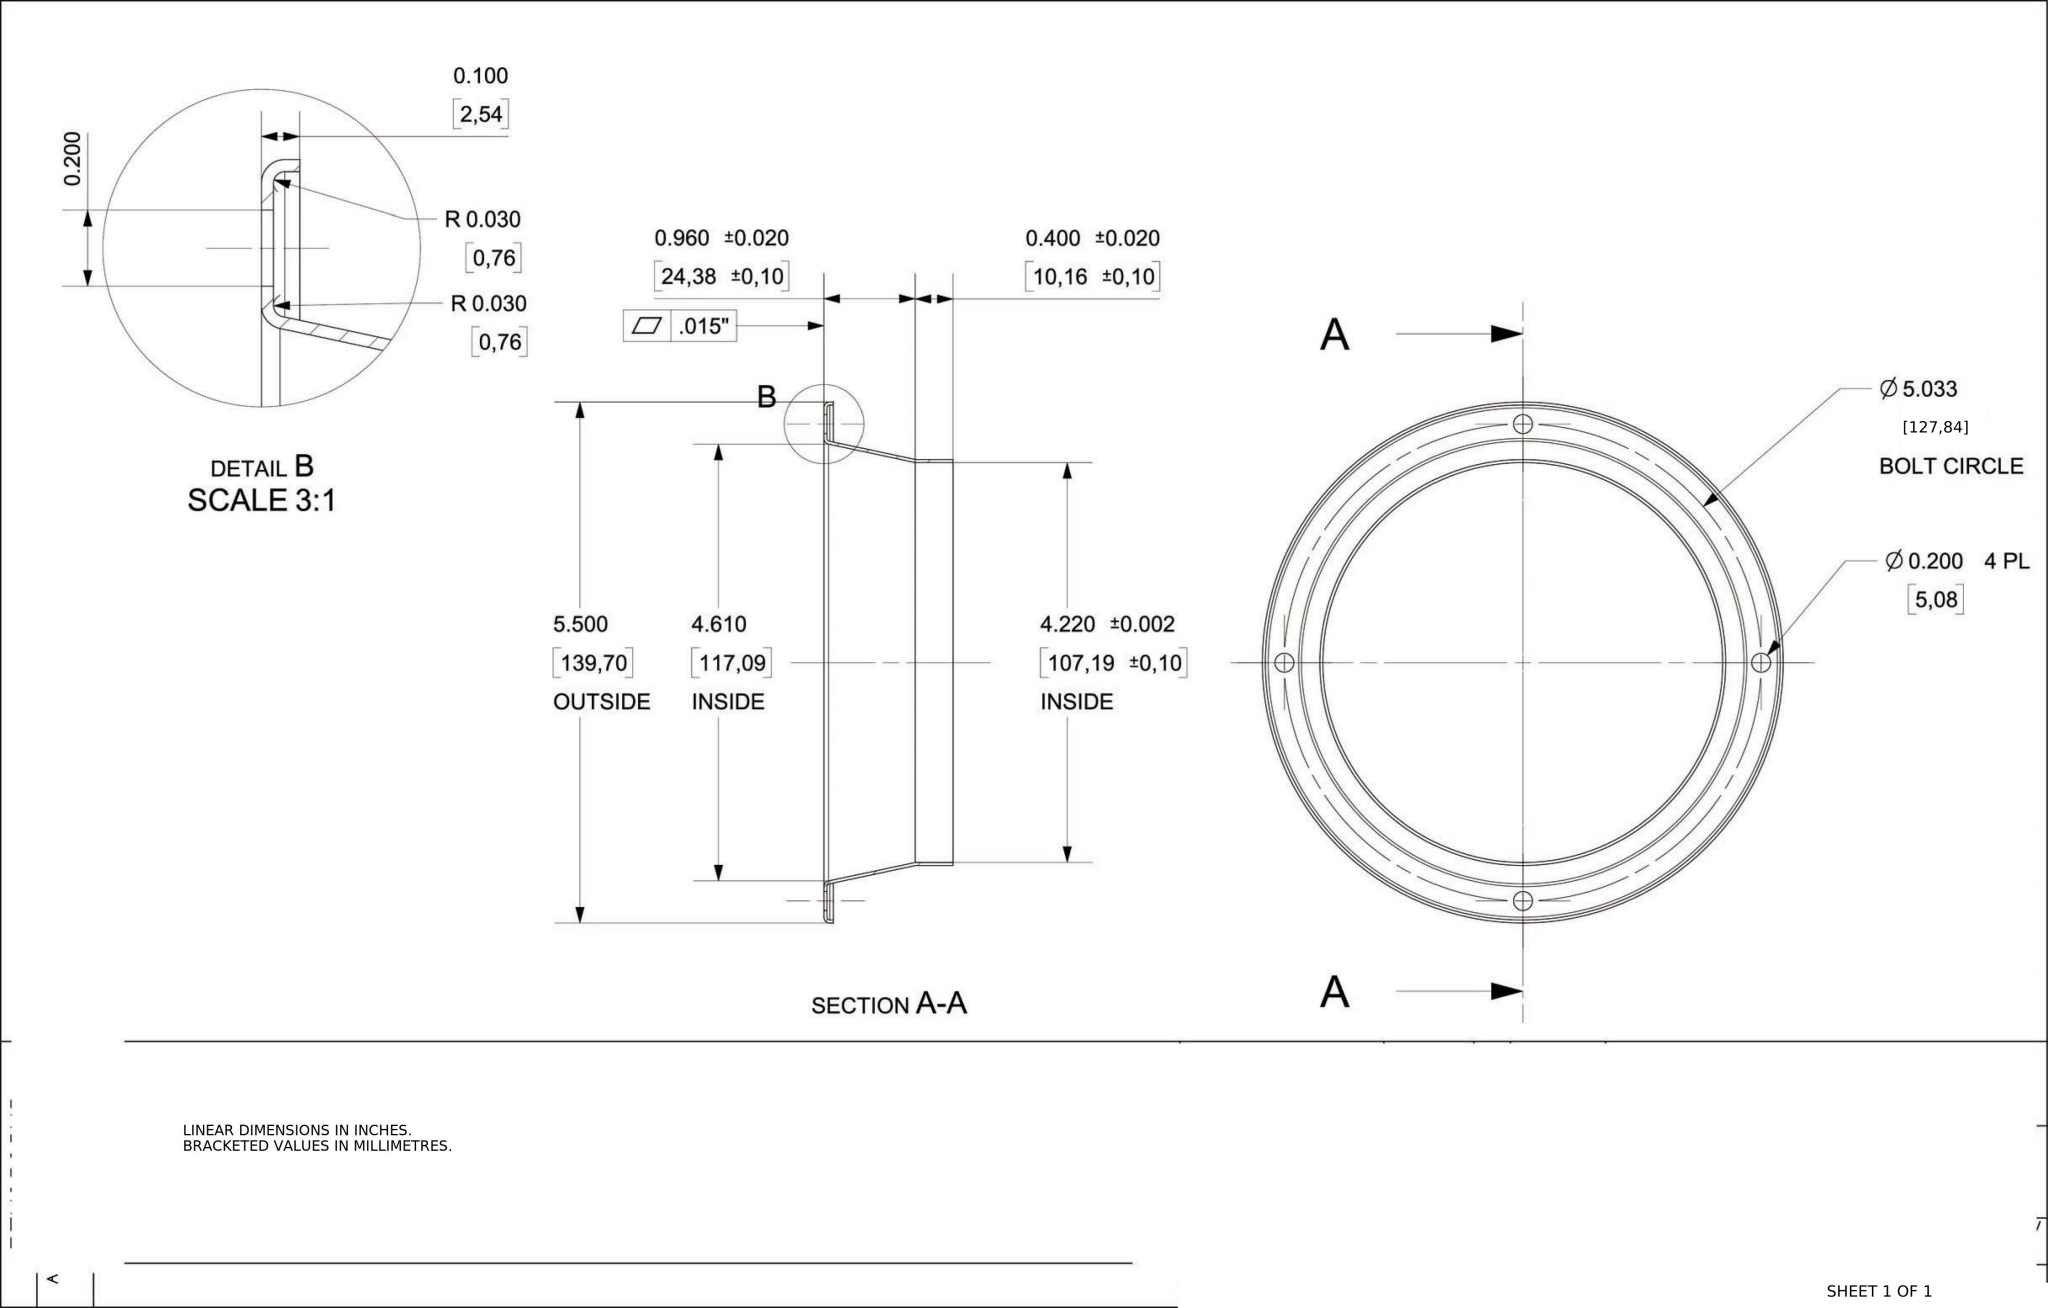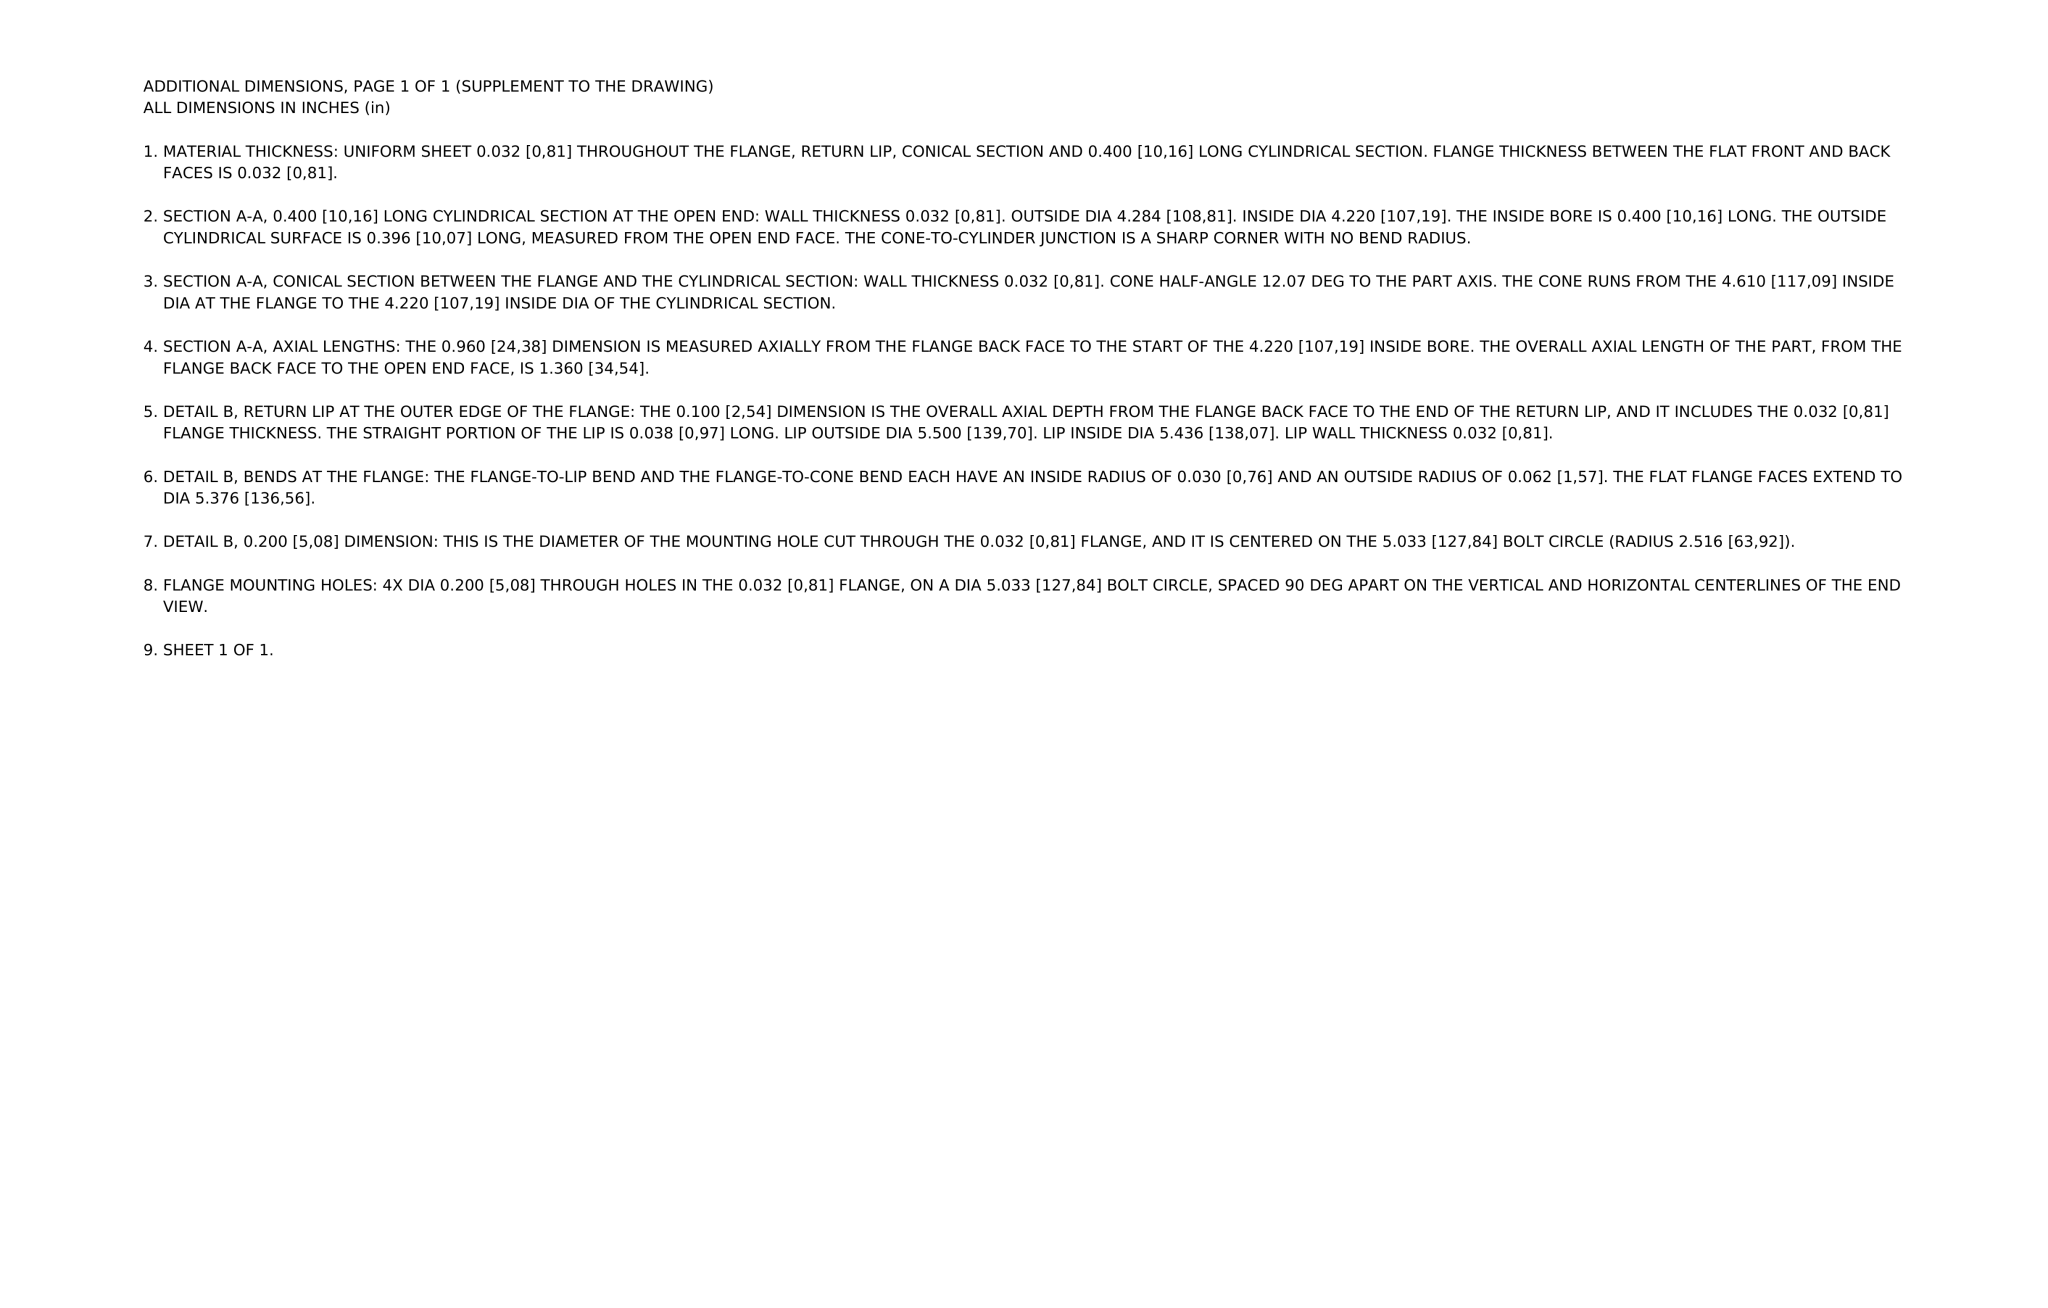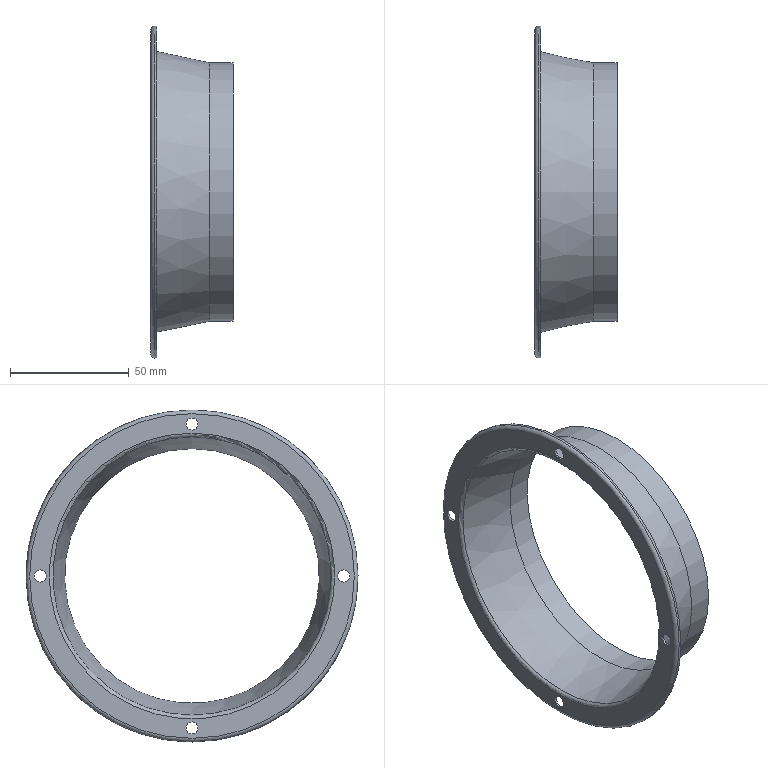Part | NX | mm | 1 solid | 18 faces | box 34.54 x 139.7 x 139.7 mm | volume 13664 mm3 | cylinder 8 | torus 4 | plane 3 | cone 3 | commonest cylinder face diameters 5.08 x4 139.7 x1 138.074 x1 108.814 x1 107.188 x1
STEP:
#1=VALUE_REPRESENTATION_ITEM('',COUNT_MEASURE(0.));
#2=(LENGTH_UNIT()NAMED_UNIT(*)SI_UNIT(.MILLI.,.METRE.));
#3=LENGTH_MEASURE_WITH_UNIT(LENGTH_MEASURE(25.4),#2);
#4=DIMENSIONAL_EXPONENTS(1.,0.,0.,0.,0.,0.,0.);
#5=(CONVERSION_BASED_UNIT('',#3)LENGTH_UNIT()NAMED_UNIT(#4));
#6=UNCERTAINTY_MEASURE_WITH_UNIT(LENGTH_MEASURE(0.002),#5,'','');
#7=(NAMED_UNIT(*)PLANE_ANGLE_UNIT()SI_UNIT($,.RADIAN.));
#8=PLANE_ANGLE_MEASURE_WITH_UNIT(PLANE_ANGLE_MEASURE(0.01745),#7);
#9=DIMENSIONAL_EXPONENTS(0.,0.,0.,0.,0.,0.,0.);
#10=(CONVERSION_BASED_UNIT('',#8)NAMED_UNIT(#9)PLANE_ANGLE_UNIT());
#11=(NAMED_UNIT(*)SI_UNIT($,.STERADIAN.)SOLID_ANGLE_UNIT());
#12=(GEOMETRIC_REPRESENTATION_CONTEXT(3)GLOBAL_UNCERTAINTY_ASSIGNED_CONTEXT((#6))GLOBAL_UNIT_ASSIGNED_CONTEXT((#5,#10,#11))REPRESENTATION_CONTEXT('',''));
#13=REPRESENTATION('',(#1),#12);
#14=VALUE_REPRESENTATION_ITEM('',COUNT_MEASURE(0.));
#15=REPRESENTATION('',(#14),#12);
#16=CARTESIAN_POINT('',(0.,0.,0.));
#17=DIRECTION('',(0.,0.,1.));
#18=DIRECTION('',(1.,0.,0.));
#19=AXIS2_PLACEMENT_3D('',#16,#17,#18);
#20=SHAPE_REPRESENTATION('',(#19),#12);
#21=CARTESIAN_POINT('',(-5.31,0.,2.688));
#22=VERTEX_POINT('',#21);
#23=CARTESIAN_POINT('',(-5.31,0.,-0.));
#24=DIRECTION('',(-1.,0.,0.));
#25=DIRECTION('',(0.,0.,1.));
#26=AXIS2_PLACEMENT_3D('',#23,#24,#25);
#27=CIRCLE('',#26,2.688);
#28=EDGE_CURVE('',#22,#22,#27,.T.);
#29=ORIENTED_EDGE('',*,*,#28,.T.);
#30=EDGE_LOOP('',(#29));
#31=FACE_BOUND('',#30,.T.);
#32=CARTESIAN_POINT('',(-5.31,0.,2.366));
#33=VERTEX_POINT('',#32);
#34=CARTESIAN_POINT('',(-5.31,0.,-0.));
#35=DIRECTION('',(1.,0.,0.));
#36=DIRECTION('',(0.,0.,1.));
#37=AXIS2_PLACEMENT_3D('',#34,#35,#36);
#38=CIRCLE('',#37,2.366);
#39=EDGE_CURVE('',#33,#33,#38,.T.);
#40=ORIENTED_EDGE('',*,*,#39,.T.);
#41=EDGE_LOOP('',(#40));
#42=FACE_BOUND('',#41,.T.);
#43=CARTESIAN_POINT('',(-5.31,-2.517,0.1));
#44=VERTEX_POINT('',#43);
#45=CARTESIAN_POINT('',(-5.31,-2.517,-0.));
#46=DIRECTION('',(-1.,0.,0.));
#47=DIRECTION('',(0.,0.,1.));
#48=AXIS2_PLACEMENT_3D('',#45,#46,#47);
#49=CIRCLE('',#48,0.1);
#50=EDGE_CURVE('',#44,#44,#49,.T.);
#51=ORIENTED_EDGE('',*,*,#50,.F.);
#52=EDGE_LOOP('',(#51));
#53=FACE_BOUND('',#52,.T.);
#54=CARTESIAN_POINT('',(-5.31,0.,2.617));
#55=VERTEX_POINT('',#54);
#56=CARTESIAN_POINT('',(-5.31,0.,2.517));
#57=DIRECTION('',(-1.,0.,0.));
#58=DIRECTION('',(0.,0.,1.));
#59=AXIS2_PLACEMENT_3D('',#56,#57,#58);
#60=CIRCLE('',#59,0.1);
#61=EDGE_CURVE('',#55,#55,#60,.T.);
#62=ORIENTED_EDGE('',*,*,#61,.F.);
#63=EDGE_LOOP('',(#62));
#64=FACE_BOUND('',#63,.T.);
#65=CARTESIAN_POINT('',(-5.31,2.517,0.1));
#66=VERTEX_POINT('',#65);
#67=CARTESIAN_POINT('',(-5.31,2.517,-0.));
#68=DIRECTION('',(-1.,0.,0.));
#69=DIRECTION('',(0.,0.,1.));
#70=AXIS2_PLACEMENT_3D('',#67,#68,#69);
#71=CIRCLE('',#70,0.1);
#72=EDGE_CURVE('',#66,#66,#71,.T.);
#73=ORIENTED_EDGE('',*,*,#72,.F.);
#74=EDGE_LOOP('',(#73));
#75=FACE_BOUND('',#74,.T.);
#76=CARTESIAN_POINT('',(-5.31,0.,-2.417));
#77=VERTEX_POINT('',#76);
#78=CARTESIAN_POINT('',(-5.31,0.,-2.517));
#79=DIRECTION('',(-1.,0.,0.));
#80=DIRECTION('',(0.,0.,1.));
#81=AXIS2_PLACEMENT_3D('',#78,#79,#80);
#82=CIRCLE('',#81,0.1);
#83=EDGE_CURVE('',#77,#77,#82,.T.);
#84=ORIENTED_EDGE('',*,*,#83,.F.);
#85=EDGE_LOOP('',(#84));
#86=FACE_BOUND('',#85,.T.);
#87=CARTESIAN_POINT('',(-5.31,0.,-2.315));
#88=DIRECTION('',(-1.,0.,0.));
#89=DIRECTION('',(0.,0.,1.));
#90=AXIS2_PLACEMENT_3D('',#87,#88,#89);
#91=PLANE('',#90);
#92=ADVANCED_FACE('',(#31,#42,#53,#64,#75,#86),#91,.T.);
#93=CARTESIAN_POINT('',(-5.248,0.,2.75));
#94=VERTEX_POINT('',#93);
#95=CARTESIAN_POINT('',(-5.248,0.,-0.));
#96=DIRECTION('',(1.,0.,0.));
#97=DIRECTION('',(0.,0.,1.));
#98=AXIS2_PLACEMENT_3D('',#95,#96,#97);
#99=CIRCLE('',#98,2.75);
#100=EDGE_CURVE('',#94,#94,#99,.T.);
#101=ORIENTED_EDGE('',*,*,#100,.T.);
#102=EDGE_LOOP('',(#101));
#103=FACE_BOUND('',#102,.T.);
#104=CARTESIAN_POINT('',(-5.21,-0.,-2.75));
#105=VERTEX_POINT('',#104);
#106=CARTESIAN_POINT('',(-5.21,0.36,-2.75));
#107=CARTESIAN_POINT('',(-5.21,-0.36,-2.75));
#108=CARTESIAN_POINT('',(-5.21,-0.7198,-2.678));
#109=CARTESIAN_POINT('',(-5.21,-1.385,-2.403));
#110=CARTESIAN_POINT('',(-5.21,-1.69,-2.199));
#111=CARTESIAN_POINT('',(-5.21,-2.199,-1.69));
#112=CARTESIAN_POINT('',(-5.21,-2.403,-1.385));
#113=CARTESIAN_POINT('',(-5.21,-2.678,-0.7198));
#114=CARTESIAN_POINT('',(-5.21,-2.75,-0.36));
#115=CARTESIAN_POINT('',(-5.21,-2.75,0.36));
#116=CARTESIAN_POINT('',(-5.21,-2.678,0.7198));
#117=CARTESIAN_POINT('',(-5.21,-2.403,1.385));
#118=CARTESIAN_POINT('',(-5.21,-2.199,1.69));
#119=CARTESIAN_POINT('',(-5.21,-1.69,2.199));
#120=CARTESIAN_POINT('',(-5.21,-1.385,2.403));
#121=CARTESIAN_POINT('',(-5.21,-0.7198,2.678));
#122=CARTESIAN_POINT('',(-5.21,-0.36,2.75));
#123=CARTESIAN_POINT('',(-5.21,0.36,2.75));
#124=CARTESIAN_POINT('',(-5.21,0.7198,2.678));
#125=CARTESIAN_POINT('',(-5.21,1.385,2.403));
#126=CARTESIAN_POINT('',(-5.21,1.69,2.199));
#127=CARTESIAN_POINT('',(-5.21,2.199,1.69));
#128=CARTESIAN_POINT('',(-5.21,2.403,1.385));
#129=CARTESIAN_POINT('',(-5.21,2.678,0.7198));
#130=CARTESIAN_POINT('',(-5.21,2.75,0.36));
#131=CARTESIAN_POINT('',(-5.21,2.75,-0.36));
#132=CARTESIAN_POINT('',(-5.21,2.678,-0.7198));
#133=CARTESIAN_POINT('',(-5.21,2.403,-1.385));
#134=CARTESIAN_POINT('',(-5.21,2.199,-1.69));
#135=CARTESIAN_POINT('',(-5.21,1.69,-2.199));
#136=CARTESIAN_POINT('',(-5.21,1.385,-2.403));
#137=CARTESIAN_POINT('',(-5.21,0.7198,-2.678));
#138=CARTESIAN_POINT('',(-5.21,0.36,-2.75));
#139=CARTESIAN_POINT('',(-5.21,-0.36,-2.75));
#140=B_SPLINE_CURVE_WITH_KNOTS('',3,(#106,#107,#108,#109,#110,#111,#112,#113,#114,#115,#116,#117,#118,#119,#120,#121,#122,#123,#124,#125,#126,#127,#128,#129,#130,#131,#132,#133,#134,#135,#136,#137,#138,#139),.UNSPECIFIED.,.T.,.F.,(2,2,2,2,2,2,2,2,2,2,2,2,2,2,2,2,2,2,2),(-0.0625,0.,0.0625,0.125,0.1875,0.25,0.3125,0.375,0.4375,0.5,0.5625,0.625,0.6875,0.75,0.8125,0.875,0.9375,1.,1.062),.UNSPECIFIED.);
#141=EDGE_CURVE('',#105,#105,#140,.T.);
#142=ORIENTED_EDGE('',*,*,#141,.T.);
#143=EDGE_LOOP('',(#142));
#144=FACE_BOUND('',#143,.T.);
#145=CARTESIAN_POINT('',(-0.28,0.,-0.));
#146=DIRECTION('',(-1.,0.,0.));
#147=DIRECTION('',(0.,0.,1.));
#148=AXIS2_PLACEMENT_3D('',#145,#146,#147);
#149=CYLINDRICAL_SURFACE('',#148,2.75);
#150=ADVANCED_FACE('',(#103,#144),#149,.T.);
#151=CARTESIAN_POINT('',(-5.21,0.,2.718));
#152=VERTEX_POINT('',#151);
#153=CARTESIAN_POINT('',(-5.21,0.,-0.));
#154=DIRECTION('',(-1.,0.,0.));
#155=DIRECTION('',(0.,0.,1.));
#156=AXIS2_PLACEMENT_3D('',#153,#154,#155);
#157=CIRCLE('',#156,2.718);
#158=EDGE_CURVE('',#152,#152,#157,.T.);
#159=ORIENTED_EDGE('',*,*,#158,.T.);
#160=EDGE_LOOP('',(#159));
#161=FACE_BOUND('',#160,.T.);
#162=ORIENTED_EDGE('',*,*,#141,.F.);
#163=EDGE_LOOP('',(#162));
#164=FACE_BOUND('',#163,.T.);
#165=CARTESIAN_POINT('',(-5.21,0.,-0.));
#166=DIRECTION('',(1.,0.,0.));
#167=DIRECTION('',(0.,0.,-1.));
#168=AXIS2_PLACEMENT_3D('',#165,#166,#167);
#169=CONICAL_SURFACE('',#168,2.75,89.597);
#170=ADVANCED_FACE('',(#161,#164),#169,.F.);
#171=CARTESIAN_POINT('',(-5.248,0.,-2.718));
#172=VERTEX_POINT('',#171);
#173=CARTESIAN_POINT('',(-5.248,0.,-0.));
#174=DIRECTION('',(-1.,0.,0.));
#175=DIRECTION('',(0.,0.,-1.));
#176=AXIS2_PLACEMENT_3D('',#173,#174,#175);
#177=CIRCLE('',#176,2.718);
#178=EDGE_CURVE('',#172,#172,#177,.T.);
#179=ORIENTED_EDGE('',*,*,#178,.T.);
#180=EDGE_LOOP('',(#179));
#181=FACE_BOUND('',#180,.T.);
#182=ORIENTED_EDGE('',*,*,#158,.F.);
#183=EDGE_LOOP('',(#182));
#184=FACE_BOUND('',#183,.T.);
#185=CARTESIAN_POINT('',(-0.28,0.,-0.));
#186=DIRECTION('',(-1.,0.,0.));
#187=DIRECTION('',(0.,0.,1.));
#188=AXIS2_PLACEMENT_3D('',#185,#186,#187);
#189=CYLINDRICAL_SURFACE('',#188,2.718);
#190=ADVANCED_FACE('',(#181,#184),#189,.F.);
#191=CARTESIAN_POINT('',(-5.278,0.,-2.688));
#192=VERTEX_POINT('',#191);
#193=CARTESIAN_POINT('',(-5.278,0.,-0.));
#194=DIRECTION('',(1.,0.,0.));
#195=DIRECTION('',(0.,0.,-1.));
#196=AXIS2_PLACEMENT_3D('',#193,#194,#195);
#197=CIRCLE('',#196,2.688);
#198=EDGE_CURVE('',#192,#192,#197,.T.);
#199=ORIENTED_EDGE('',*,*,#198,.T.);
#200=EDGE_LOOP('',(#199));
#201=FACE_BOUND('',#200,.T.);
#202=CARTESIAN_POINT('',(-5.278,-2.517,0.1));
#203=VERTEX_POINT('',#202);
#204=CARTESIAN_POINT('',(-5.278,-2.517,-0.));
#205=DIRECTION('',(-1.,0.,0.));
#206=DIRECTION('',(0.,0.,1.));
#207=AXIS2_PLACEMENT_3D('',#204,#205,#206);
#208=CIRCLE('',#207,0.1);
#209=EDGE_CURVE('',#203,#203,#208,.T.);
#210=ORIENTED_EDGE('',*,*,#209,.T.);
#211=EDGE_LOOP('',(#210));
#212=FACE_BOUND('',#211,.T.);
#213=CARTESIAN_POINT('',(-5.278,0.,2.617));
#214=VERTEX_POINT('',#213);
#215=CARTESIAN_POINT('',(-5.278,0.,2.517));
#216=DIRECTION('',(-1.,0.,0.));
#217=DIRECTION('',(0.,0.,1.));
#218=AXIS2_PLACEMENT_3D('',#215,#216,#217);
#219=CIRCLE('',#218,0.1);
#220=EDGE_CURVE('',#214,#214,#219,.T.);
#221=ORIENTED_EDGE('',*,*,#220,.T.);
#222=EDGE_LOOP('',(#221));
#223=FACE_BOUND('',#222,.T.);
#224=CARTESIAN_POINT('',(-5.278,2.517,0.1));
#225=VERTEX_POINT('',#224);
#226=CARTESIAN_POINT('',(-5.278,2.517,-0.));
#227=DIRECTION('',(-1.,0.,0.));
#228=DIRECTION('',(0.,0.,1.));
#229=AXIS2_PLACEMENT_3D('',#226,#227,#228);
#230=CIRCLE('',#229,0.1);
#231=EDGE_CURVE('',#225,#225,#230,.T.);
#232=ORIENTED_EDGE('',*,*,#231,.T.);
#233=EDGE_LOOP('',(#232));
#234=FACE_BOUND('',#233,.T.);
#235=CARTESIAN_POINT('',(-5.278,0.,-2.417));
#236=VERTEX_POINT('',#235);
#237=CARTESIAN_POINT('',(-5.278,0.,-2.517));
#238=DIRECTION('',(-1.,0.,0.));
#239=DIRECTION('',(0.,0.,1.));
#240=AXIS2_PLACEMENT_3D('',#237,#238,#239);
#241=CIRCLE('',#240,0.1);
#242=EDGE_CURVE('',#236,#236,#241,.T.);
#243=ORIENTED_EDGE('',*,*,#242,.T.);
#244=EDGE_LOOP('',(#243));
#245=FACE_BOUND('',#244,.T.);
#246=CARTESIAN_POINT('',(-5.278,0.,2.366));
#247=VERTEX_POINT('',#246);
#248=CARTESIAN_POINT('',(-5.278,0.,-0.));
#249=DIRECTION('',(-1.,0.,0.));
#250=DIRECTION('',(0.,0.,1.));
#251=AXIS2_PLACEMENT_3D('',#248,#249,#250);
#252=CIRCLE('',#251,2.366);
#253=EDGE_CURVE('',#247,#247,#252,.T.);
#254=ORIENTED_EDGE('',*,*,#253,.T.);
#255=EDGE_LOOP('',(#254));
#256=FACE_BOUND('',#255,.T.);
#257=CARTESIAN_POINT('',(-5.278,0.,-2.718));
#258=DIRECTION('',(1.,0.,0.));
#259=DIRECTION('',(0.,0.,-1.));
#260=AXIS2_PLACEMENT_3D('',#257,#258,#259);
#261=PLANE('',#260);
#262=ADVANCED_FACE('',(#201,#212,#223,#234,#245,#256),#261,.T.);
#263=CARTESIAN_POINT('',(-5.254,0.,2.336));
#264=VERTEX_POINT('',#263);
#265=CARTESIAN_POINT('',(-5.254,0.,-0.));
#266=DIRECTION('',(-1.,0.,0.));
#267=DIRECTION('',(0.,0.,1.));
#268=AXIS2_PLACEMENT_3D('',#265,#266,#267);
#269=CIRCLE('',#268,2.336);
#270=EDGE_CURVE('',#264,#264,#269,.T.);
#271=ORIENTED_EDGE('',*,*,#270,.T.);
#272=EDGE_LOOP('',(#271));
#273=FACE_BOUND('',#272,.T.);
#274=ORIENTED_EDGE('',*,*,#253,.F.);
#275=EDGE_LOOP('',(#274));
#276=FACE_BOUND('',#275,.T.);
#277=CARTESIAN_POINT('',(-5.248,0.,-0.));
#278=DIRECTION('',(-1.,0.,0.));
#279=DIRECTION('',(0.,0.,1.));
#280=AXIS2_PLACEMENT_3D('',#277,#278,#279);
#281=TOROIDAL_SURFACE('',#280,2.366,0.03);
#282=ADVANCED_FACE('',(#273,#276),#281,.F.);
#283=CARTESIAN_POINT('',(-4.347,0.,2.142));
#284=VERTEX_POINT('',#283);
#285=CARTESIAN_POINT('',(-4.347,0.,-0.));
#286=DIRECTION('',(-1.,0.,0.));
#287=DIRECTION('',(0.,0.,1.));
#288=AXIS2_PLACEMENT_3D('',#285,#286,#287);
#289=CIRCLE('',#288,2.142);
#290=EDGE_CURVE('',#284,#284,#289,.T.);
#291=ORIENTED_EDGE('',*,*,#290,.T.);
#292=EDGE_LOOP('',(#291));
#293=FACE_BOUND('',#292,.T.);
#294=ORIENTED_EDGE('',*,*,#270,.F.);
#295=EDGE_LOOP('',(#294));
#296=FACE_BOUND('',#295,.T.);
#297=CARTESIAN_POINT('',(-5.254,0.,-0.));
#298=DIRECTION('',(-1.,0.,0.));
#299=DIRECTION('',(-0.,0.,1.));
#300=AXIS2_PLACEMENT_3D('',#297,#298,#299);
#301=CONICAL_SURFACE('',#300,2.336,12.075);
#302=ADVANCED_FACE('',(#293,#296),#301,.T.);
#303=CARTESIAN_POINT('',(-3.95,0.,2.142));
#304=VERTEX_POINT('',#303);
#305=CARTESIAN_POINT('',(-3.95,0.,-0.));
#306=DIRECTION('',(-1.,0.,0.));
#307=DIRECTION('',(0.,0.,1.));
#308=AXIS2_PLACEMENT_3D('',#305,#306,#307);
#309=CIRCLE('',#308,2.142);
#310=EDGE_CURVE('',#304,#304,#309,.T.);
#311=ORIENTED_EDGE('',*,*,#310,.T.);
#312=EDGE_LOOP('',(#311));
#313=FACE_BOUND('',#312,.T.);
#314=ORIENTED_EDGE('',*,*,#290,.F.);
#315=EDGE_LOOP('',(#314));
#316=FACE_BOUND('',#315,.T.);
#317=CARTESIAN_POINT('',(-0.28,0.,-0.));
#318=DIRECTION('',(-1.,0.,0.));
#319=DIRECTION('',(0.,0.,1.));
#320=AXIS2_PLACEMENT_3D('',#317,#318,#319);
#321=CYLINDRICAL_SURFACE('',#320,2.142);
#322=ADVANCED_FACE('',(#313,#316),#321,.T.);
#323=CARTESIAN_POINT('',(-3.95,0.,2.11));
#324=VERTEX_POINT('',#323);
#325=CARTESIAN_POINT('',(-3.95,0.,-0.));
#326=DIRECTION('',(-1.,0.,0.));
#327=DIRECTION('',(0.,0.,1.));
#328=AXIS2_PLACEMENT_3D('',#325,#326,#327);
#329=CIRCLE('',#328,2.11);
#330=EDGE_CURVE('',#324,#324,#329,.T.);
#331=ORIENTED_EDGE('',*,*,#330,.T.);
#332=EDGE_LOOP('',(#331));
#333=FACE_BOUND('',#332,.T.);
#334=ORIENTED_EDGE('',*,*,#310,.F.);
#335=EDGE_LOOP('',(#334));
#336=FACE_BOUND('',#335,.T.);
#337=CARTESIAN_POINT('',(-3.95,0.,-2.142));
#338=DIRECTION('',(1.,0.,0.));
#339=DIRECTION('',(0.,0.,-1.));
#340=AXIS2_PLACEMENT_3D('',#337,#338,#339);
#341=PLANE('',#340);
#342=ADVANCED_FACE('',(#333,#336),#341,.T.);
#343=CARTESIAN_POINT('',(-4.35,0.,2.11));
#344=VERTEX_POINT('',#343);
#345=CARTESIAN_POINT('',(-4.35,0.,-0.));
#346=DIRECTION('',(-1.,0.,0.));
#347=DIRECTION('',(0.,0.,1.));
#348=AXIS2_PLACEMENT_3D('',#345,#346,#347);
#349=CIRCLE('',#348,2.11);
#350=EDGE_CURVE('',#344,#344,#349,.T.);
#351=ORIENTED_EDGE('',*,*,#350,.T.);
#352=EDGE_LOOP('',(#351));
#353=FACE_BOUND('',#352,.T.);
#354=ORIENTED_EDGE('',*,*,#330,.F.);
#355=EDGE_LOOP('',(#354));
#356=FACE_BOUND('',#355,.T.);
#357=CARTESIAN_POINT('',(-0.28,0.,-0.));
#358=DIRECTION('',(-1.,0.,0.));
#359=DIRECTION('',(0.,0.,1.));
#360=AXIS2_PLACEMENT_3D('',#357,#358,#359);
#361=CYLINDRICAL_SURFACE('',#360,2.11);
#362=ADVANCED_FACE('',(#353,#356),#361,.F.);
#363=CARTESIAN_POINT('',(-5.261,0.,-2.305));
#364=VERTEX_POINT('',#363);
#365=CARTESIAN_POINT('',(-5.261,0.,-0.));
#366=DIRECTION('',(-1.,0.,0.));
#367=DIRECTION('',(0.,0.,-1.));
#368=AXIS2_PLACEMENT_3D('',#365,#366,#367);
#369=CIRCLE('',#368,2.305);
#370=EDGE_CURVE('',#364,#364,#369,.T.);
#371=ORIENTED_EDGE('',*,*,#370,.T.);
#372=EDGE_LOOP('',(#371));
#373=FACE_BOUND('',#372,.T.);
#374=ORIENTED_EDGE('',*,*,#350,.F.);
#375=EDGE_LOOP('',(#374));
#376=FACE_BOUND('',#375,.T.);
#377=CARTESIAN_POINT('',(-4.35,0.,-0.));
#378=DIRECTION('',(-1.,0.,0.));
#379=DIRECTION('',(0.,0.,1.));
#380=AXIS2_PLACEMENT_3D('',#377,#378,#379);
#381=CONICAL_SURFACE('',#380,2.11,12.075);
#382=ADVANCED_FACE('',(#373,#376),#381,.F.);
#383=ORIENTED_EDGE('',*,*,#83,.T.);
#384=EDGE_LOOP('',(#383));
#385=FACE_BOUND('',#384,.T.);
#386=ORIENTED_EDGE('',*,*,#242,.F.);
#387=EDGE_LOOP('',(#386));
#388=FACE_BOUND('',#387,.T.);
#389=CARTESIAN_POINT('',(-5.278,0.,-2.517));
#390=DIRECTION('',(-1.,0.,0.));
#391=DIRECTION('',(0.,0.,1.));
#392=AXIS2_PLACEMENT_3D('',#389,#390,#391);
#393=CYLINDRICAL_SURFACE('',#392,0.1);
#394=ADVANCED_FACE('',(#385,#388),#393,.F.);
#395=ORIENTED_EDGE('',*,*,#72,.T.);
#396=EDGE_LOOP('',(#395));
#397=FACE_BOUND('',#396,.T.);
#398=ORIENTED_EDGE('',*,*,#231,.F.);
#399=EDGE_LOOP('',(#398));
#400=FACE_BOUND('',#399,.T.);
#401=CARTESIAN_POINT('',(-5.278,2.517,-0.));
#402=DIRECTION('',(-1.,0.,0.));
#403=DIRECTION('',(0.,0.,1.));
#404=AXIS2_PLACEMENT_3D('',#401,#402,#403);
#405=CYLINDRICAL_SURFACE('',#404,0.1);
#406=ADVANCED_FACE('',(#397,#400),#405,.F.);
#407=ORIENTED_EDGE('',*,*,#61,.T.);
#408=EDGE_LOOP('',(#407));
#409=FACE_BOUND('',#408,.T.);
#410=ORIENTED_EDGE('',*,*,#220,.F.);
#411=EDGE_LOOP('',(#410));
#412=FACE_BOUND('',#411,.T.);
#413=CARTESIAN_POINT('',(-5.278,0.,2.517));
#414=DIRECTION('',(-1.,0.,0.));
#415=DIRECTION('',(0.,0.,1.));
#416=AXIS2_PLACEMENT_3D('',#413,#414,#415);
#417=CYLINDRICAL_SURFACE('',#416,0.1);
#418=ADVANCED_FACE('',(#409,#412),#417,.F.);
#419=ORIENTED_EDGE('',*,*,#50,.T.);
#420=EDGE_LOOP('',(#419));
#421=FACE_BOUND('',#420,.T.);
#422=ORIENTED_EDGE('',*,*,#209,.F.);
#423=EDGE_LOOP('',(#422));
#424=FACE_BOUND('',#423,.T.);
#425=CARTESIAN_POINT('',(-5.278,-2.517,-0.));
#426=DIRECTION('',(-1.,0.,0.));
#427=DIRECTION('',(0.,0.,1.));
#428=AXIS2_PLACEMENT_3D('',#425,#426,#427);
#429=CYLINDRICAL_SURFACE('',#428,0.1);
#430=ADVANCED_FACE('',(#421,#424),#429,.F.);
#431=ORIENTED_EDGE('',*,*,#39,.F.);
#432=EDGE_LOOP('',(#431));
#433=FACE_BOUND('',#432,.T.);
#434=ORIENTED_EDGE('',*,*,#370,.F.);
#435=EDGE_LOOP('',(#434));
#436=FACE_BOUND('',#435,.T.);
#437=CARTESIAN_POINT('',(-5.248,0.,-0.));
#438=DIRECTION('',(-1.,0.,0.));
#439=DIRECTION('',(0.,0.,1.));
#440=AXIS2_PLACEMENT_3D('',#437,#438,#439);
#441=TOROIDAL_SURFACE('',#440,2.366,0.062);
#442=ADVANCED_FACE('',(#433,#436),#441,.T.);
#443=ORIENTED_EDGE('',*,*,#198,.F.);
#444=EDGE_LOOP('',(#443));
#445=FACE_BOUND('',#444,.T.);
#446=ORIENTED_EDGE('',*,*,#178,.F.);
#447=EDGE_LOOP('',(#446));
#448=FACE_BOUND('',#447,.T.);
#449=CARTESIAN_POINT('',(-5.248,0.,-0.));
#450=DIRECTION('',(1.,0.,0.));
#451=DIRECTION('',(0.,0.,-1.));
#452=AXIS2_PLACEMENT_3D('',#449,#450,#451);
#453=TOROIDAL_SURFACE('',#452,2.688,0.03);
#454=ADVANCED_FACE('',(#445,#448),#453,.F.);
#455=ORIENTED_EDGE('',*,*,#100,.F.);
#456=EDGE_LOOP('',(#455));
#457=FACE_BOUND('',#456,.T.);
#458=ORIENTED_EDGE('',*,*,#28,.F.);
#459=EDGE_LOOP('',(#458));
#460=FACE_BOUND('',#459,.T.);
#461=CARTESIAN_POINT('',(-5.248,0.,-0.));
#462=DIRECTION('',(-1.,0.,0.));
#463=DIRECTION('',(0.,0.,1.));
#464=AXIS2_PLACEMENT_3D('',#461,#462,#463);
#465=TOROIDAL_SURFACE('',#464,2.688,0.062);
#466=ADVANCED_FACE('',(#457,#460),#465,.T.);
#467=CLOSED_SHELL('',(#92,#150,#170,#190,#262,#282,#302,#322,#342,#362,#382,#394,#406,#418,#430,#442,#454,#466));
#468=MANIFOLD_SOLID_BREP('',#467);
#469=ADVANCED_BREP_SHAPE_REPRESENTATION('',(#468),#12);
#470=SHAPE_REPRESENTATION_RELATIONSHIP('','',#20,#469);